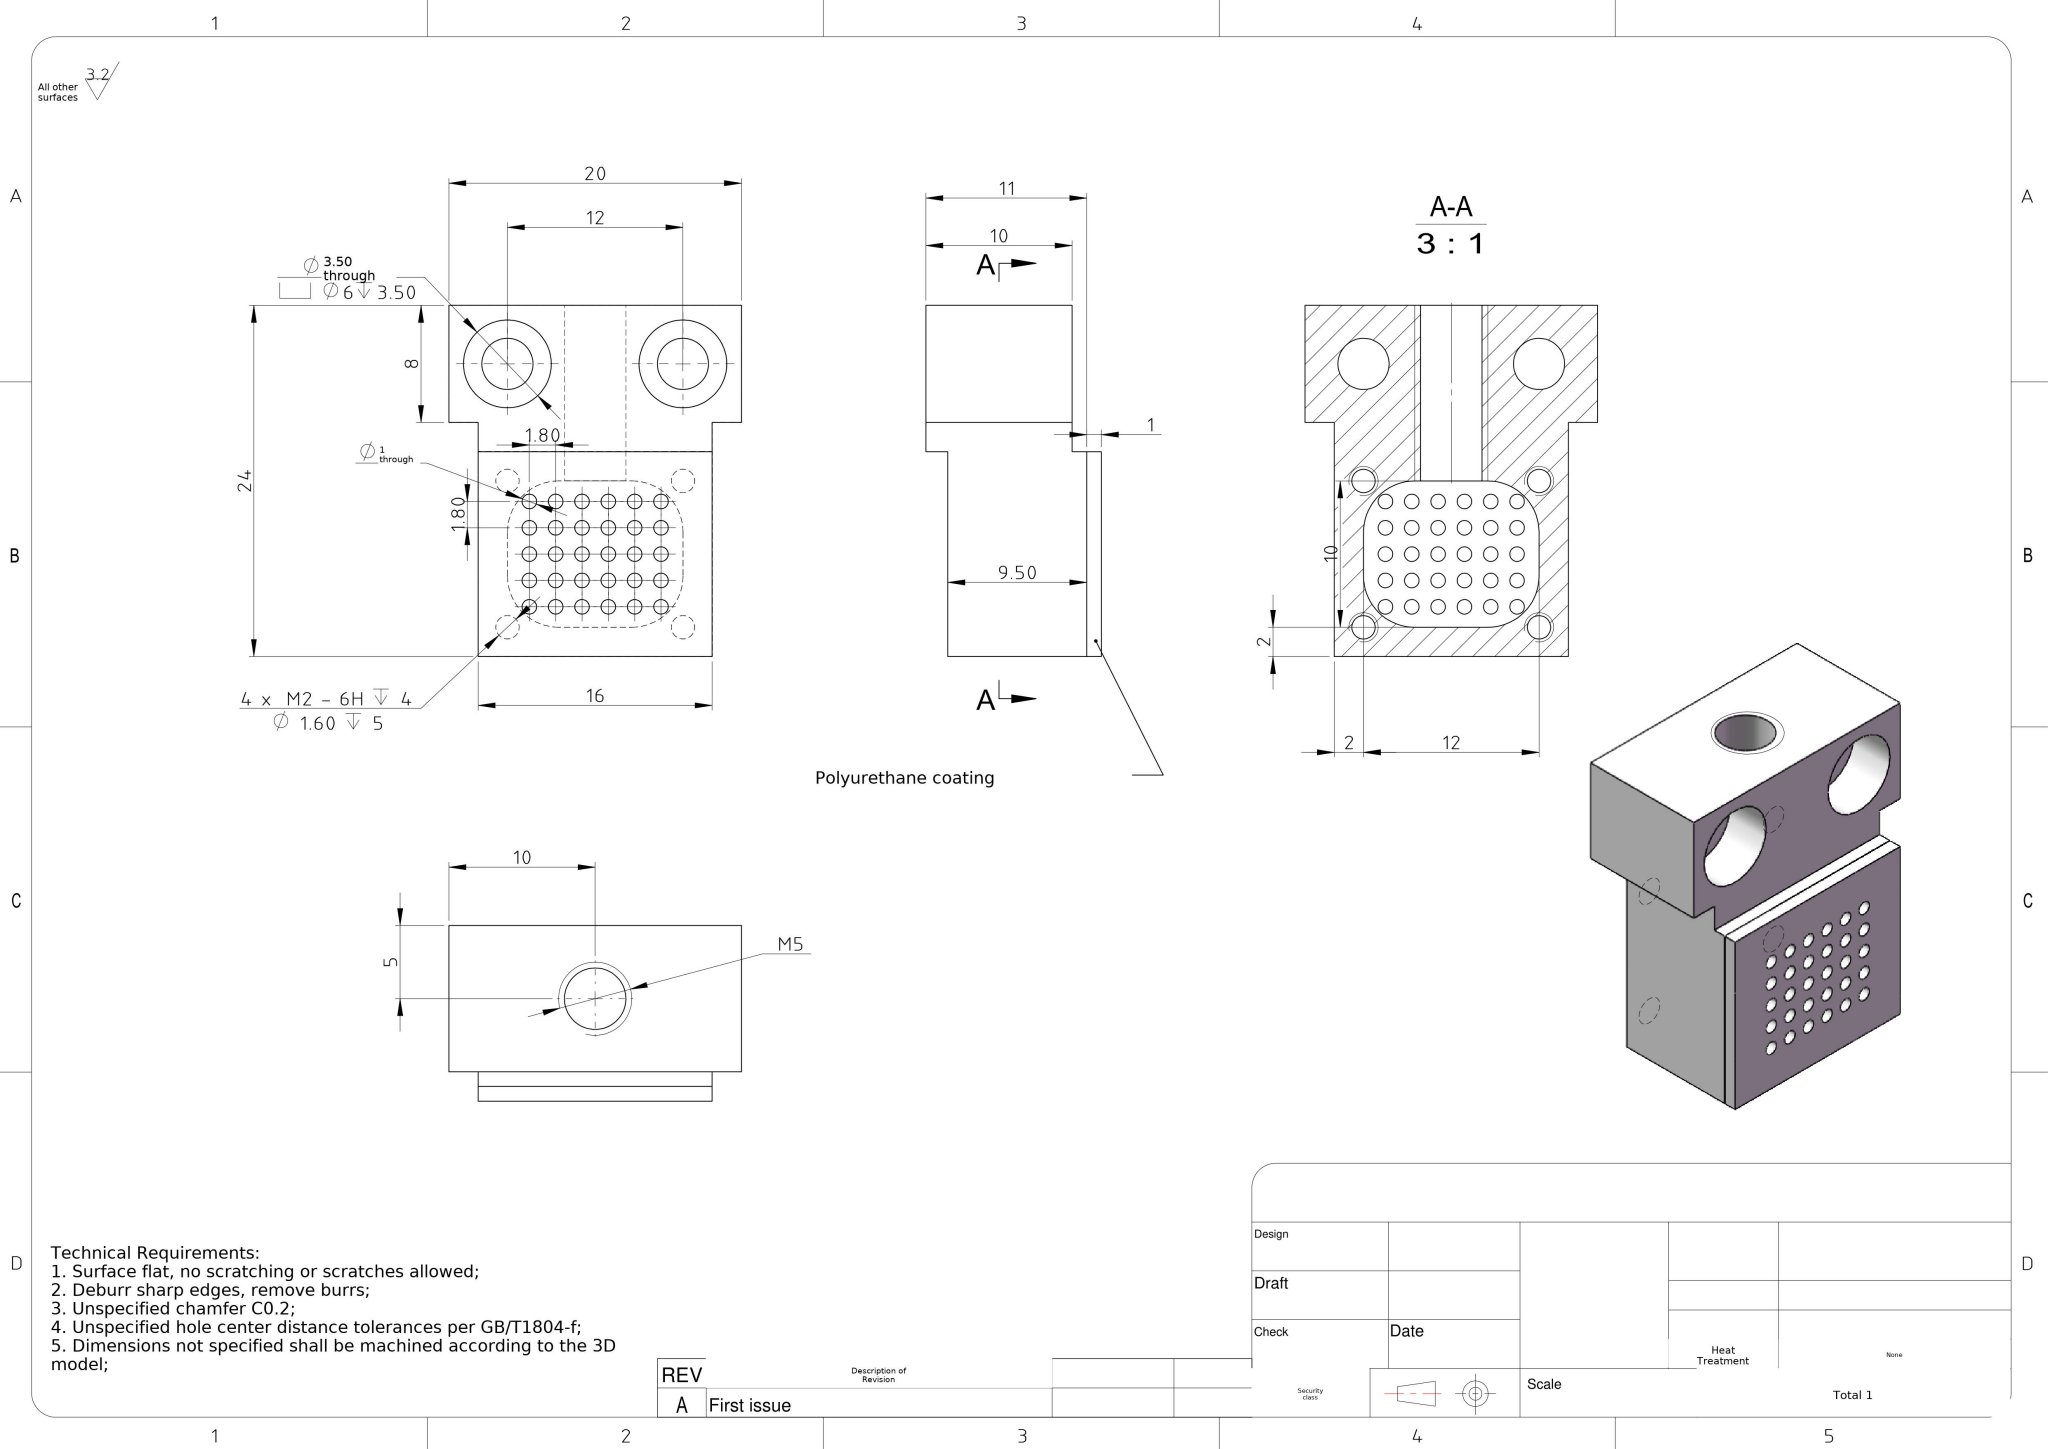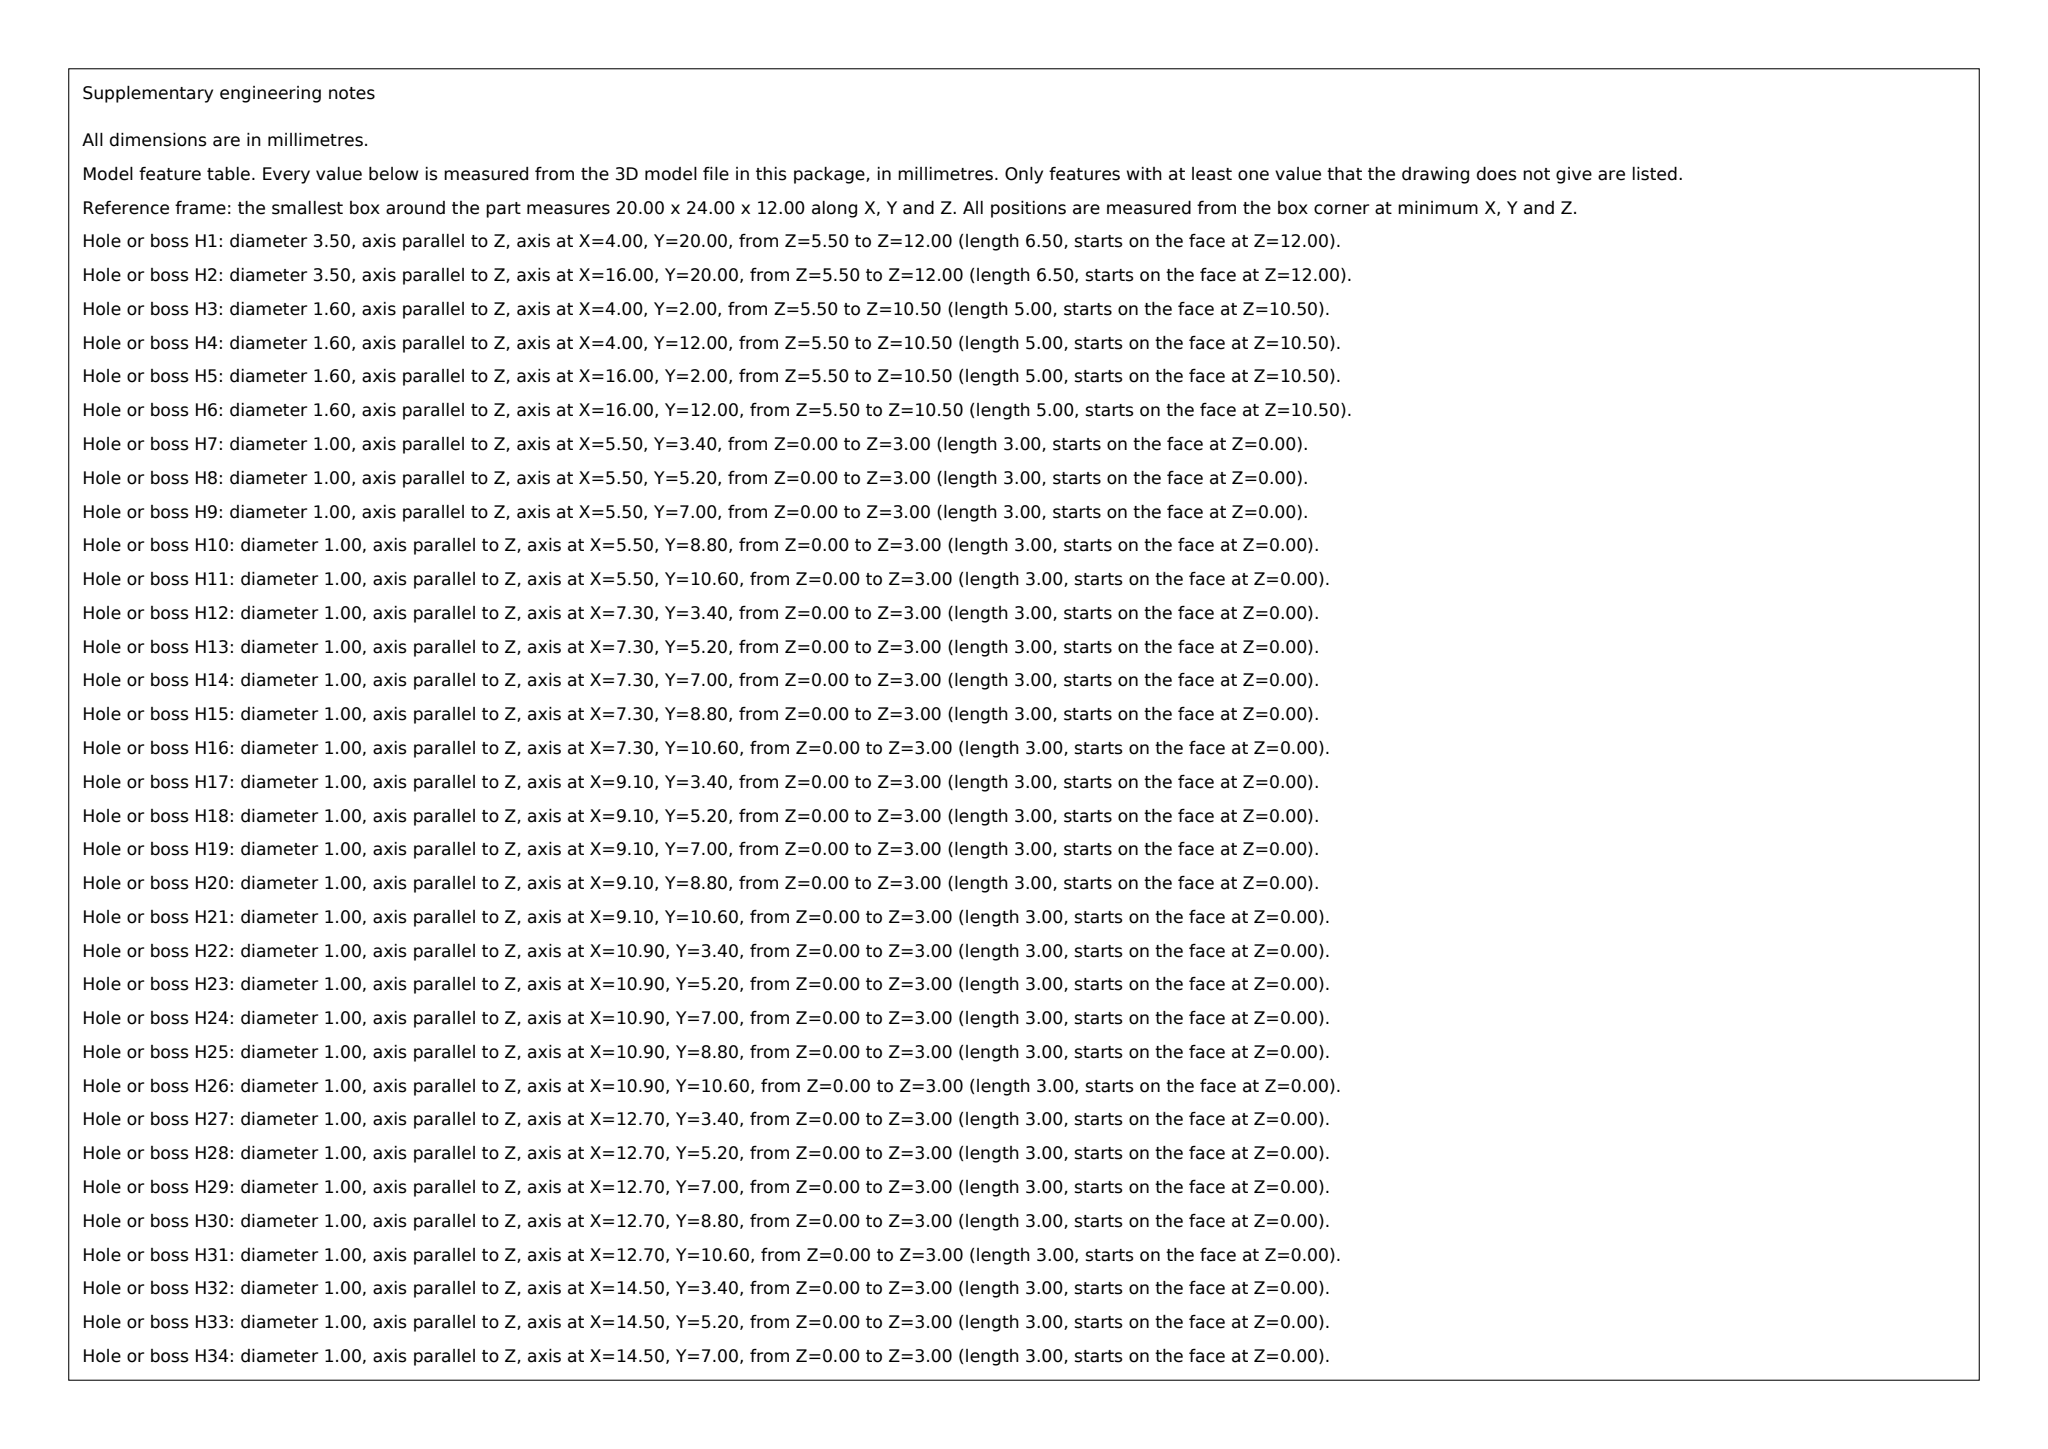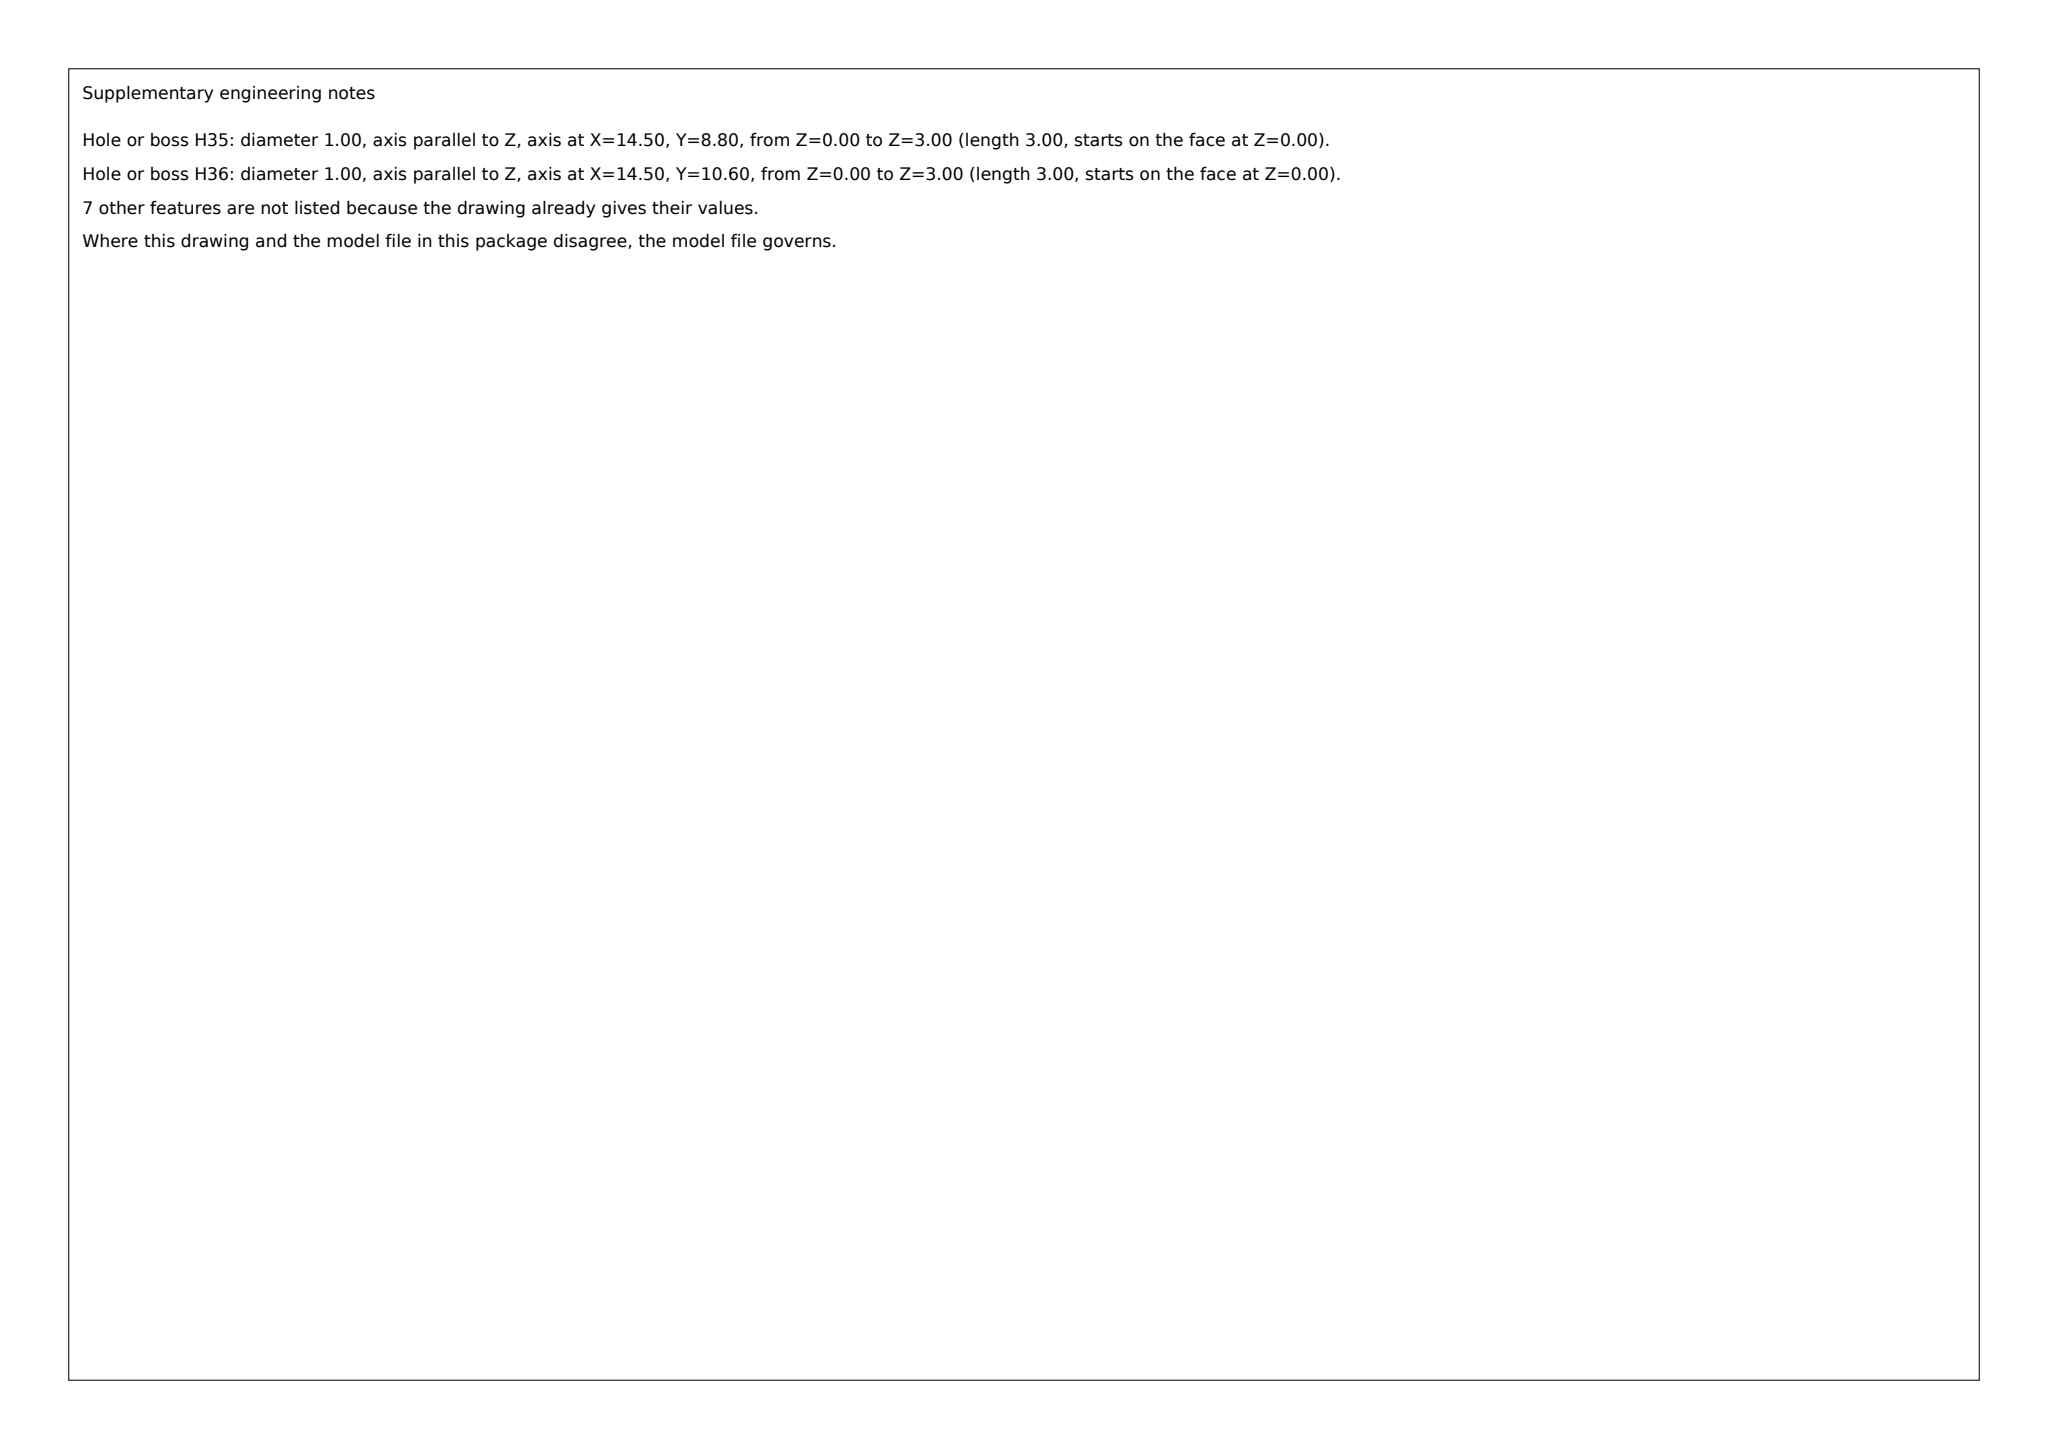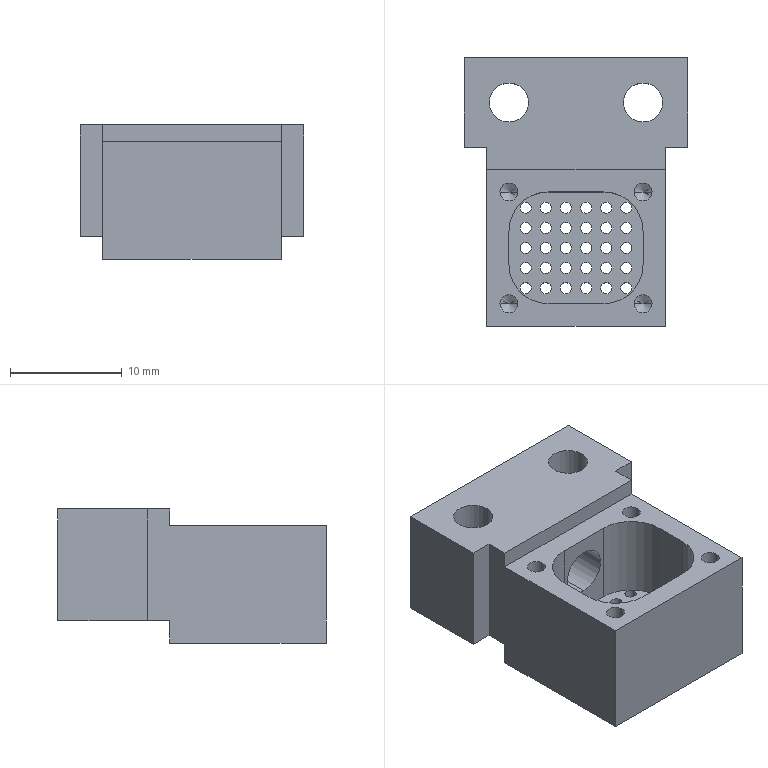Part | SolidWorks | mm | 1 solid | 111 faces | box 20 x 24 x 12 mm | volume 2849 mm3 | cylinder 82 | plane 21 | cone 8 | commonest cylinder face diameters 1 x60 1.6 x8 6 x4 3.5 x4 7 x4 4.2 x2
build123d program:
from build123d import *

# Parameters (mm, degrees)
SKETCH1_W            = 16
SKETCH1_H            = 24
BOSS_EXTRUDE4_DEPTH  = 10
SKETCH21_W           = 12
SKETCH21_H           = 10
CUT_EXTRUDE3_DEPTH   = 9
SKETCH22_W           = 16
SKETCH22_H           = 14
BOSS_EXTRUDE5_DEPTH  = 1
SKETCH34_W           = 16
SKETCH34_H           = 14
BOSS_EXTRUDE8_DEPTH  = 1
FILLET2_R            = 3.5
SKETCH23_R           = 0.5
CUT_EXTRUDE4_DEPTH   = 18
LPATTERN1_COUNT      = 6
LPATTERN1_PITCH      = 1.8
LPATTERN1_COUNT_DIR2 = 5
LPATTERN1_PITCH_DIR2 = 1.8
SKETCH25_W           = 2.1
SKETCH25_H           = 12
SKETCH26_W           = 16
SKETCH26_H           = 14
CUT_EXTRUDE5_DEPTH   = 1.5
SKETCH29_W           = 2
SKETCH29_H           = 10
BOSS_EXTRUDE7_DEPTH  = 10
SKETCH27_R           = 1.75
CUT_EXTRUDE7_DEPTH   = 19.547
SKETCH28_R           = 3
CUT_EXTRUDE8_DEPTH   = 3.5
SKETCH35_W           = 2
SKETCH35_H           = 2
CUT_EXTRUDE10_DEPTH  = 20.698
LPATTERN2_COUNT      = 2
LPATTERN2_PITCH      = 10
LPATTERN2_COUNT_DIR2 = 2
LPATTERN2_PITCH_DIR2 = 12
SKETCH36_R           = 0.5
CUT_EXTRUDE11_DEPTH  = 20.105


with BuildPart() as part:
    # Sketch1 → Boss-Extrude4 (new body)
    with BuildSketch(Plane.XY):
        Rectangle(SKETCH1_W, SKETCH1_H)
    extrude(amount=BOSS_EXTRUDE4_DEPTH)

    # Sketch21 → Cut-Extrude3 (cut)
    with BuildSketch(Plane.XY.offset(10)):
        with Locations((0, -5)):
            Rectangle(SKETCH21_W, SKETCH21_H)
    extrude(amount=-CUT_EXTRUDE3_DEPTH, mode=Mode.SUBTRACT)

    # Sketch22 → Boss-Extrude5 (add)
    with BuildSketch(Plane(origin=(0, 0, 0), x_dir=(-1, 0, 0), z_dir=(0, 0, -1))):
        with Locations((0, -5)):
            Rectangle(SKETCH22_W, SKETCH22_H)
    extrude(amount=BOSS_EXTRUDE5_DEPTH)

    # Fillet2
    fillet2_edges = [part.edges().sort_by_distance(p)[0] for p in [
        (-6, -10, 5.5),
        (-6, 0, 5.5),
        (6, 0, 5.5),
        (6, -10, 5.5),
    ]]
    fillet(fillet2_edges, radius=FILLET2_R)

    # Sketch23 → Cut-Extrude4 (cut, through all)
    with BuildSketch(Plane.XY.offset(1)):
        with Locations((-4.5, -8.6)):
            Circle(SKETCH23_R)
    cut_extrude4 = extrude(amount=-CUT_EXTRUDE4_DEPTH, mode=Mode.SUBTRACT)

    # LPattern1: Cut-Extrude4 6 × 5
    with Locations(*[(i * LPATTERN1_PITCH, j * LPATTERN1_PITCH_DIR2, 0) for i in range(LPATTERN1_COUNT) for j in range(LPATTERN1_COUNT_DIR2) if (i, j) != (0, 0)]):
        add(cut_extrude4, mode=Mode.SUBTRACT)

    # Sketch25 → M5 Tapped Hole1 (revolve, cut)
    with BuildSketch(Plane(origin=(0, 12, 5), x_dir=(0, 0, 1), z_dir=(1, 0, 0))):
        with Locations((1.05, 6)):
            Rectangle(SKETCH25_W, SKETCH25_H)
    revolve(axis=Axis((0, 18.35, 5), (0, -1, 0)), mode=Mode.SUBTRACT)

    # Sketch26 → Cut-Extrude5 (cut)
    with BuildSketch(Plane.XY.offset(10)):
        with Locations((0, -5)):
            Rectangle(SKETCH26_W, SKETCH26_H)
    extrude(amount=-CUT_EXTRUDE5_DEPTH, mode=Mode.SUBTRACT)

    # Sketch29 → Boss-Extrude7 (add)
    with BuildSketch(Plane.XY.offset(10)):
        with Locations((9, 7)):
            Rectangle(SKETCH29_W, SKETCH29_H)
        with Locations((-9, 7)):
            Rectangle(SKETCH29_W, SKETCH29_H)
    extrude(amount=-BOSS_EXTRUDE7_DEPTH)

    # Sketch27 → Cut-Extrude7 (cut, through all)
    with BuildSketch(Plane(origin=(0, 0, 0), x_dir=(-1, 0, 0), z_dir=(0, 0, -1))):
        with Locations((-6, 8)):
            Circle(SKETCH27_R)
        with Locations(Location((6, 8, 0), (0, 0, 180))):
            Circle(SKETCH27_R)
    extrude(amount=-CUT_EXTRUDE7_DEPTH, mode=Mode.SUBTRACT)

    # Sketch28 → Cut-Extrude8 (cut)
    with BuildSketch(Plane(origin=(0, 0, 0), x_dir=(-1, 0, 0), z_dir=(0, 0, -1))):
        with Locations((-6, 8)):
            Circle(SKETCH28_R)
        with Locations((6, 8)):
            Circle(SKETCH28_R)
    extrude(amount=-CUT_EXTRUDE8_DEPTH, mode=Mode.SUBTRACT)

    # Sketch35 → Cut-Extrude10 (cut, through all)
    with BuildSketch(Plane.XY.offset(10)):
        with Locations((-9, 3)):
            Rectangle(SKETCH35_W, SKETCH35_H)
        with Locations((9, 3)):
            Rectangle(SKETCH35_W, SKETCH35_H)
    extrude(amount=-CUT_EXTRUDE10_DEPTH, mode=Mode.SUBTRACT)

    # Sketch31 → M2 Tapped Hole1 (revolve, cut)
    with BuildSketch(Plane(origin=(6, -10, 8.5), x_dir=(0, -1, 0), z_dir=(1, 0, 0))):
        Polygon((0, 0), (0, 5.481), (0.8, 5), (0.8, 0), align=None)
    m2_tapped_hole1 = revolve(axis=Axis((6, -10, 14.85), (0, 0, -1)), mode=Mode.SUBTRACT)

    # LPattern2: M2 Tapped Hole1 2 × 2
    with Locations(*[(-j * LPATTERN2_PITCH_DIR2, i * LPATTERN2_PITCH, 0) for i in range(LPATTERN2_COUNT) for j in range(LPATTERN2_COUNT_DIR2) if (i, j) != (0, 0)]):
        add(m2_tapped_hole1, mode=Mode.SUBTRACT)


with BuildPart() as body_2:
    # Sketch34 → Boss-Extrude8 (new body)
    with BuildSketch(Plane(origin=(0, 0, -1), x_dir=(-1, 0, 0), z_dir=(0, 0, -1))):
        with Locations((0, -5)):
            Rectangle(SKETCH34_W, SKETCH34_H)
    extrude(amount=BOSS_EXTRUDE8_DEPTH)

    # Sketch36 → Cut-Extrude11 (cut, through all)
    with BuildSketch(Plane.XY.offset(-1)):
        with Locations((-4.5, -8.6)):
            Circle(SKETCH36_R)
        with Locations((-2.7, -8.6)):
            Circle(SKETCH36_R)
        with Locations((-0.9, -8.6)):
            Circle(SKETCH36_R)
        with Locations((0.9, -8.6)):
            Circle(SKETCH36_R)
        with Locations((2.7, -8.6)):
            Circle(SKETCH36_R)
        with Locations((-2.7, -6.8)):
            Circle(SKETCH36_R)
        with Locations((-0.9, -6.8)):
            Circle(SKETCH36_R)
        with Locations((0.9, -6.8)):
            Circle(SKETCH36_R)
        with Locations((2.7, -6.8)):
            Circle(SKETCH36_R)
        with Locations((-2.7, -5)):
            Circle(SKETCH36_R)
        with Locations((-0.9, -5)):
            Circle(SKETCH36_R)
        with Locations((0.9, -5)):
            Circle(SKETCH36_R)
        with Locations((2.7, -5)):
            Circle(SKETCH36_R)
        with Locations((-2.7, -3.2)):
            Circle(SKETCH36_R)
        with Locations((-0.9, -3.2)):
            Circle(SKETCH36_R)
        with Locations((0.9, -3.2)):
            Circle(SKETCH36_R)
        with Locations((2.7, -3.2)):
            Circle(SKETCH36_R)
        with Locations((-4.5, -6.8)):
            Circle(SKETCH36_R)
        with Locations((-4.5, -5)):
            Circle(SKETCH36_R)
        with Locations((-4.5, -3.2)):
            Circle(SKETCH36_R)
        with Locations((4.5, -8.6)):
            Circle(SKETCH36_R)
        with Locations((4.5, -6.8)):
            Circle(SKETCH36_R)
        with Locations((4.5, -5)):
            Circle(SKETCH36_R)
        with Locations((4.5, -3.2)):
            Circle(SKETCH36_R)
        with Locations((-4.5, -1.4)):
            Circle(SKETCH36_R)
        with Locations((-2.7, -1.4)):
            Circle(SKETCH36_R)
        with Locations((-0.9, -1.4)):
            Circle(SKETCH36_R)
        with Locations((0.9, -1.4)):
            Circle(SKETCH36_R)
        with Locations((2.7, -1.4)):
            Circle(SKETCH36_R)
        with Locations((4.5, -1.4)):
            Circle(SKETCH36_R)
    extrude(amount=-CUT_EXTRUDE11_DEPTH, mode=Mode.SUBTRACT)

    # Combine-RayDong-Repair: union part
    add(part.part)


solid = body_2.part